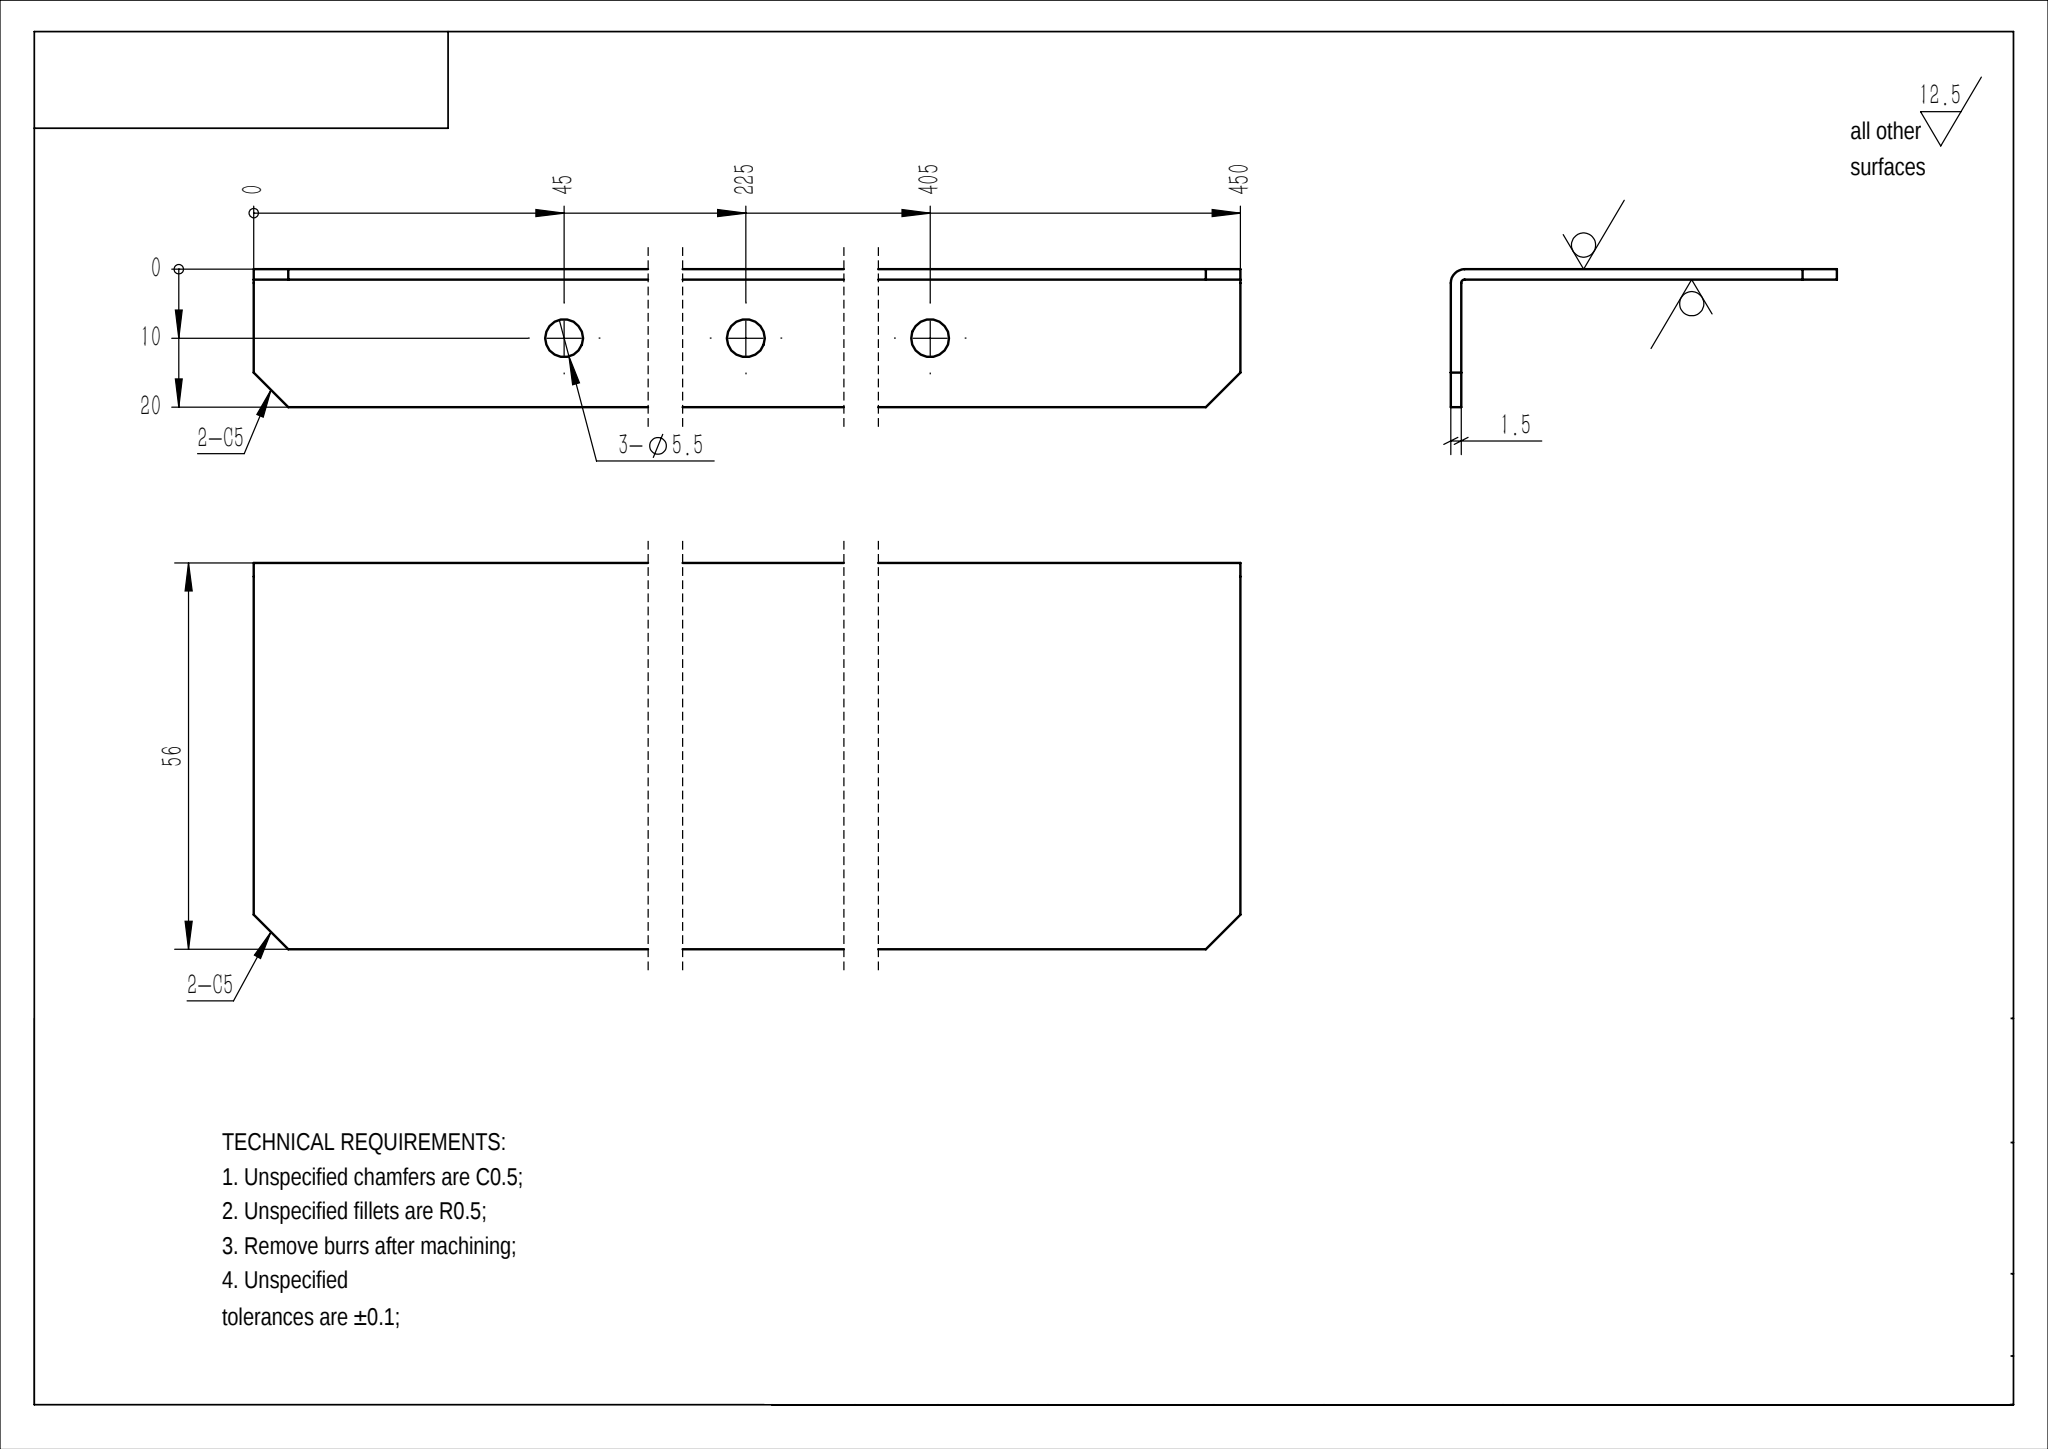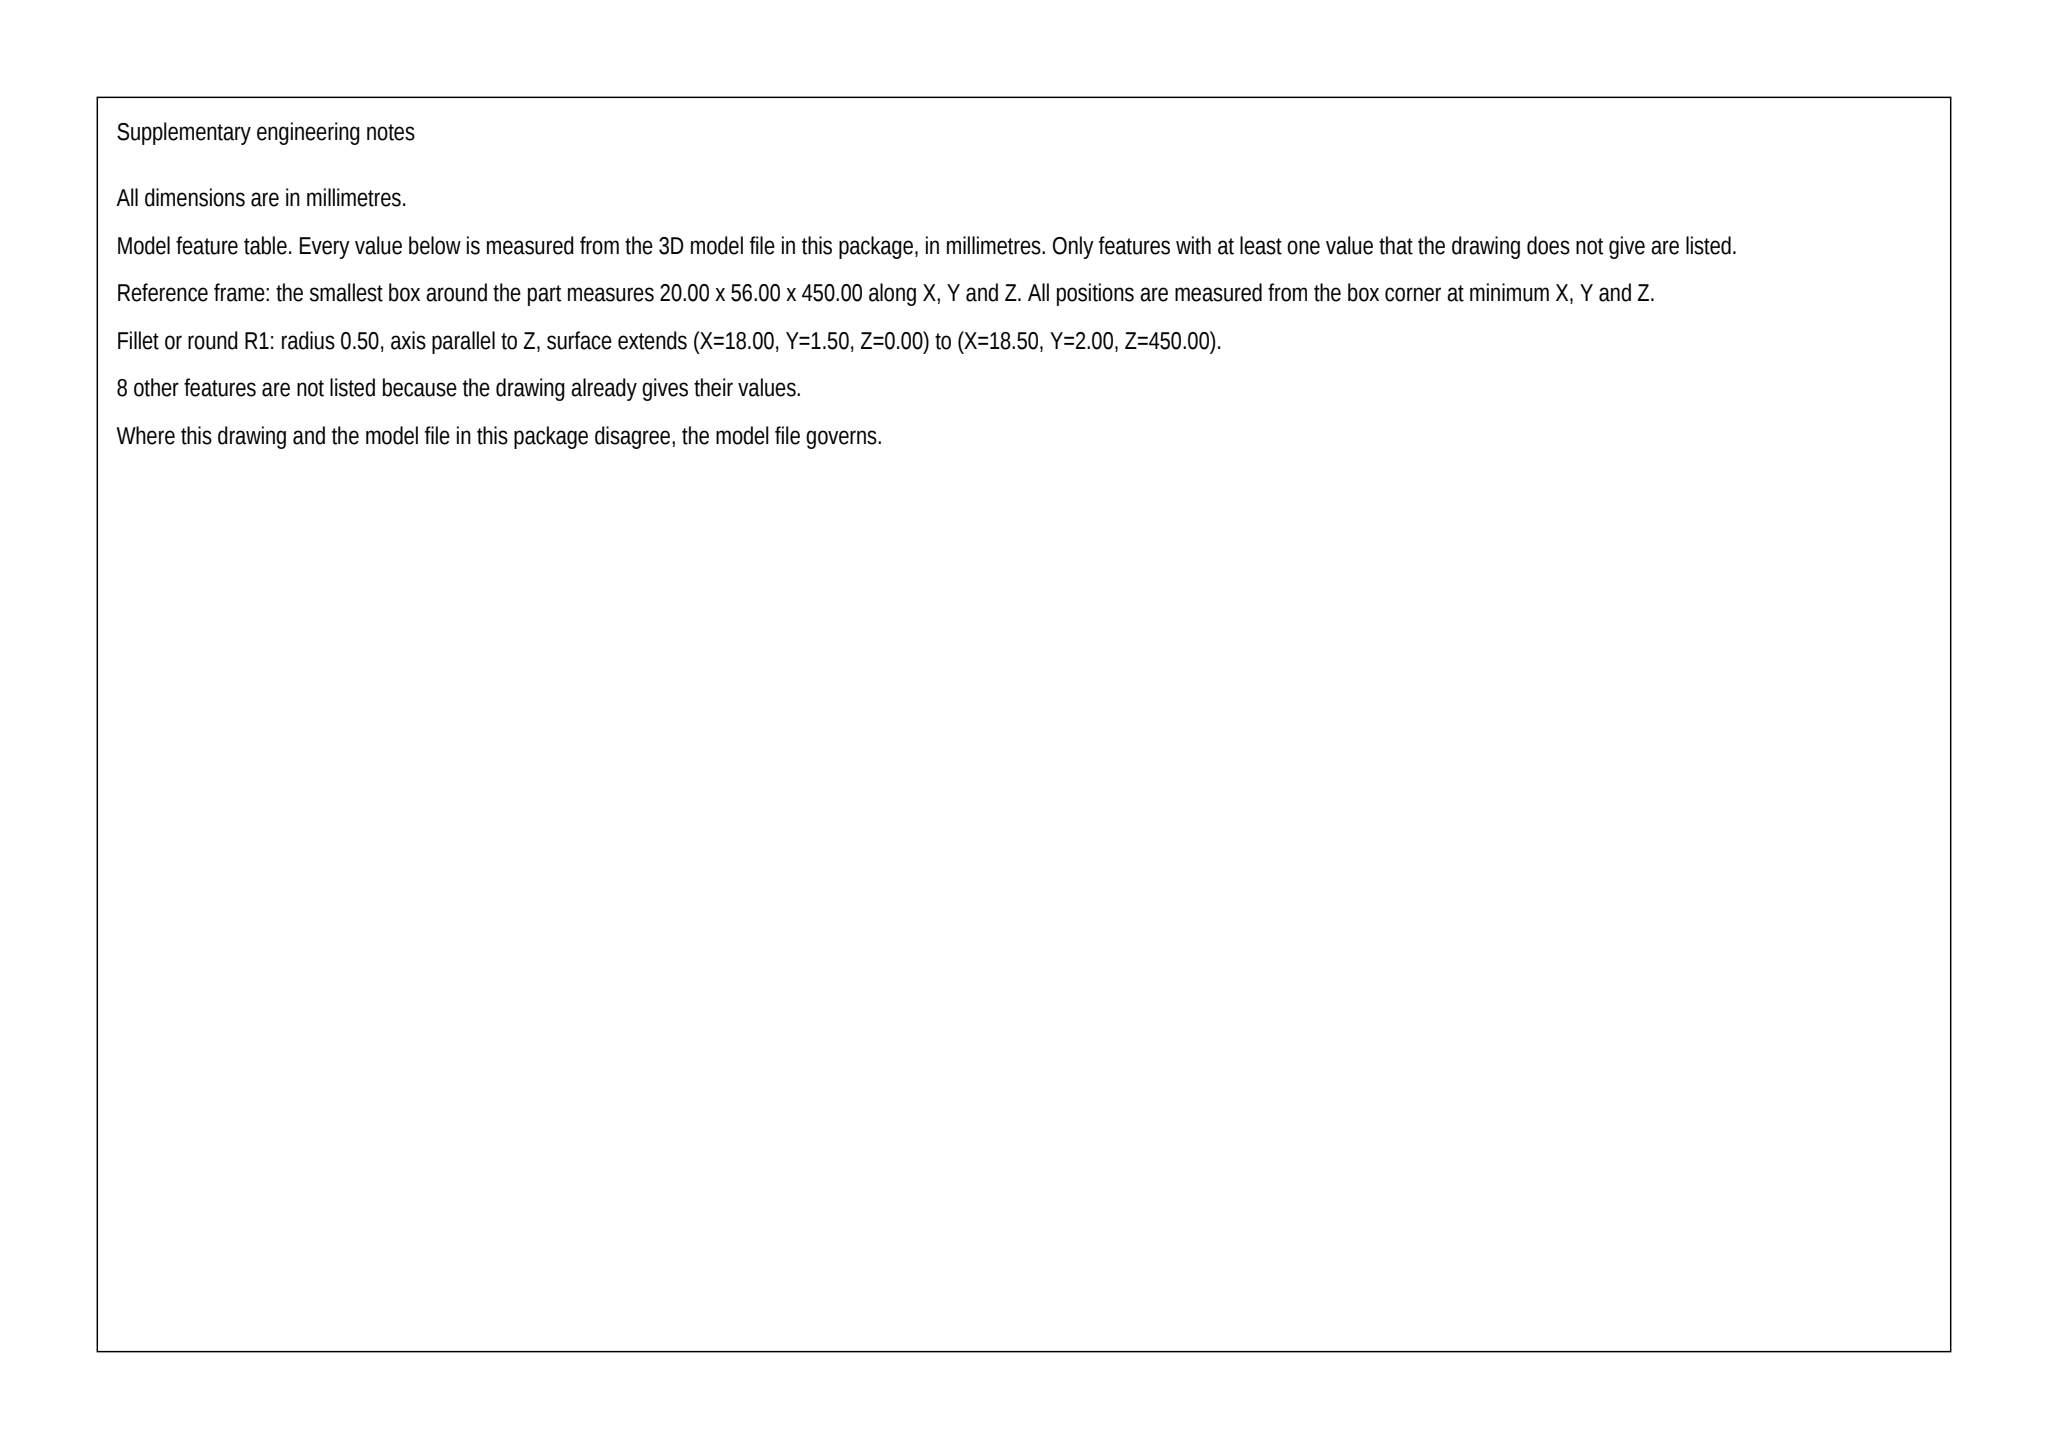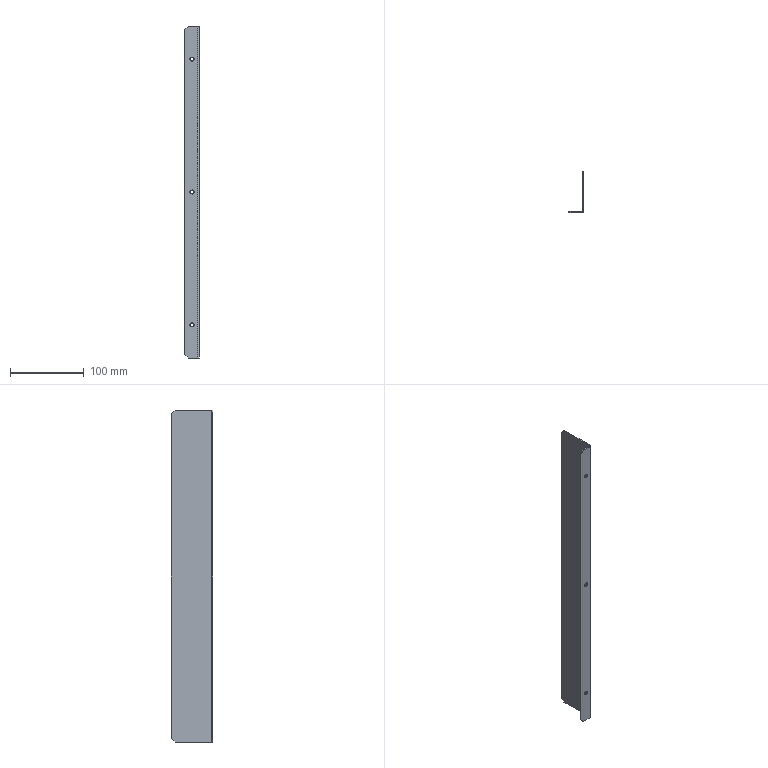Part | SolidWorks | mm | 1 solid | 24 faces | box 20 x 56 x 450 mm | volume 49743 mm3 | plane 16 | cylinder 8 | commonest cylinder face diameters 5.5 x6 1 x1 4 x1
STEP:
#1=CARTESIAN_POINT('',(-8.5,-1.5,-2.75));
#2=VERTEX_POINT('',#1);
#3=CARTESIAN_POINT('',(-8.5,-1.5,2.75));
#4=VERTEX_POINT('',#3);
#5=CARTESIAN_POINT('',(-8.5,-1.5,0.));
#6=DIRECTION('',(0.,1.,0.));
#7=DIRECTION('',(0.,0.,1.));
#8=AXIS2_PLACEMENT_3D('',#5,#6,#7);
#9=CIRCLE('',#8,2.75);
#10=EDGE_CURVE('',#2,#4,#9,.T.);
#11=ORIENTED_EDGE('',*,*,#10,.F.);
#12=CARTESIAN_POINT('',(-8.5,0.,-2.75));
#13=VERTEX_POINT('',#12);
#14=CARTESIAN_POINT('',(-8.5,-1.5,-2.75));
#15=DIRECTION('',(0.,1.,0.));
#16=VECTOR('',#15,1000.);
#17=LINE('',#14,#16);
#18=EDGE_CURVE('',#2,#13,#17,.T.);
#19=ORIENTED_EDGE('',*,*,#18,.T.);
#20=CARTESIAN_POINT('',(-8.5,0.,2.75));
#21=VERTEX_POINT('',#20);
#22=CARTESIAN_POINT('',(-8.5,0.,0.));
#23=DIRECTION('',(0.,1.,0.));
#24=DIRECTION('',(0.,0.,1.));
#25=AXIS2_PLACEMENT_3D('',#22,#23,#24);
#26=CIRCLE('',#25,2.75);
#27=EDGE_CURVE('',#13,#21,#26,.T.);
#28=ORIENTED_EDGE('',*,*,#27,.T.);
#29=CARTESIAN_POINT('',(-8.5,-1.5,2.75));
#30=DIRECTION('',(0.,1.,0.));
#31=VECTOR('',#30,1000.);
#32=LINE('',#29,#31);
#33=EDGE_CURVE('',#4,#21,#32,.T.);
#34=ORIENTED_EDGE('',*,*,#33,.F.);
#35=EDGE_LOOP('',(#11,#19,#28,#34));
#36=FACE_OUTER_BOUND('',#35,.T.);
#37=CARTESIAN_POINT('',(-8.5,-1.5,0.));
#38=DIRECTION('',(0.,1.,0.));
#39=DIRECTION('',(0.,0.,1.));
#40=AXIS2_PLACEMENT_3D('',#37,#38,#39);
#41=CYLINDRICAL_SURFACE('',#40,2.75);
#42=ADVANCED_FACE('',(#36),#41,.F.);
#43=CARTESIAN_POINT('',(-8.5,-1.5,177.25));
#44=VERTEX_POINT('',#43);
#45=CARTESIAN_POINT('',(-8.5,-1.5,182.75));
#46=VERTEX_POINT('',#45);
#47=CARTESIAN_POINT('',(-8.5,-1.5,180.));
#48=DIRECTION('',(0.,1.,0.));
#49=DIRECTION('',(0.,0.,-1.));
#50=AXIS2_PLACEMENT_3D('',#47,#48,#49);
#51=CIRCLE('',#50,2.75);
#52=EDGE_CURVE('',#44,#46,#51,.T.);
#53=ORIENTED_EDGE('',*,*,#52,.F.);
#54=CARTESIAN_POINT('',(-8.5,0.,177.25));
#55=VERTEX_POINT('',#54);
#56=CARTESIAN_POINT('',(-8.5,-1.5,177.25));
#57=DIRECTION('',(0.,1.,0.));
#58=VECTOR('',#57,1000.);
#59=LINE('',#56,#58);
#60=EDGE_CURVE('',#44,#55,#59,.T.);
#61=ORIENTED_EDGE('',*,*,#60,.T.);
#62=CARTESIAN_POINT('',(-8.5,0.,182.75));
#63=VERTEX_POINT('',#62);
#64=CARTESIAN_POINT('',(-8.5,0.,180.));
#65=DIRECTION('',(0.,1.,0.));
#66=DIRECTION('',(0.,0.,-1.));
#67=AXIS2_PLACEMENT_3D('',#64,#65,#66);
#68=CIRCLE('',#67,2.75);
#69=EDGE_CURVE('',#55,#63,#68,.T.);
#70=ORIENTED_EDGE('',*,*,#69,.T.);
#71=CARTESIAN_POINT('',(-8.5,-1.5,182.75));
#72=DIRECTION('',(0.,1.,0.));
#73=VECTOR('',#72,1000.);
#74=LINE('',#71,#73);
#75=EDGE_CURVE('',#46,#63,#74,.T.);
#76=ORIENTED_EDGE('',*,*,#75,.F.);
#77=EDGE_LOOP('',(#53,#61,#70,#76));
#78=FACE_OUTER_BOUND('',#77,.T.);
#79=CARTESIAN_POINT('',(-8.5,-1.5,180.));
#80=DIRECTION('',(0.,1.,0.));
#81=DIRECTION('',(0.,0.,1.));
#82=AXIS2_PLACEMENT_3D('',#79,#80,#81);
#83=CYLINDRICAL_SURFACE('',#82,2.75);
#84=ADVANCED_FACE('',(#78),#83,.F.);
#85=CARTESIAN_POINT('',(-8.5,-1.5,-182.75));
#86=VERTEX_POINT('',#85);
#87=CARTESIAN_POINT('',(-8.5,-1.5,-177.25));
#88=VERTEX_POINT('',#87);
#89=CARTESIAN_POINT('',(-8.5,-1.5,-180.));
#90=DIRECTION('',(0.,1.,0.));
#91=DIRECTION('',(0.,0.,1.));
#92=AXIS2_PLACEMENT_3D('',#89,#90,#91);
#93=CIRCLE('',#92,2.75);
#94=EDGE_CURVE('',#86,#88,#93,.T.);
#95=ORIENTED_EDGE('',*,*,#94,.F.);
#96=CARTESIAN_POINT('',(-8.5,0.,-182.75));
#97=VERTEX_POINT('',#96);
#98=CARTESIAN_POINT('',(-8.5,-1.5,-182.75));
#99=DIRECTION('',(0.,1.,0.));
#100=VECTOR('',#99,1000.);
#101=LINE('',#98,#100);
#102=EDGE_CURVE('',#86,#97,#101,.T.);
#103=ORIENTED_EDGE('',*,*,#102,.T.);
#104=CARTESIAN_POINT('',(-8.5,0.,-177.25));
#105=VERTEX_POINT('',#104);
#106=CARTESIAN_POINT('',(-8.5,0.,-180.));
#107=DIRECTION('',(0.,1.,0.));
#108=DIRECTION('',(0.,0.,1.));
#109=AXIS2_PLACEMENT_3D('',#106,#107,#108);
#110=CIRCLE('',#109,2.75);
#111=EDGE_CURVE('',#97,#105,#110,.T.);
#112=ORIENTED_EDGE('',*,*,#111,.T.);
#113=CARTESIAN_POINT('',(-8.5,-1.5,-177.25));
#114=DIRECTION('',(0.,1.,0.));
#115=VECTOR('',#114,1000.);
#116=LINE('',#113,#115);
#117=EDGE_CURVE('',#88,#105,#116,.T.);
#118=ORIENTED_EDGE('',*,*,#117,.F.);
#119=EDGE_LOOP('',(#95,#103,#112,#118));
#120=FACE_OUTER_BOUND('',#119,.T.);
#121=CARTESIAN_POINT('',(-8.5,-1.5,-180.));
#122=DIRECTION('',(0.,1.,0.));
#123=DIRECTION('',(0.,0.,1.));
#124=AXIS2_PLACEMENT_3D('',#121,#122,#123);
#125=CYLINDRICAL_SURFACE('',#124,2.75);
#126=ADVANCED_FACE('',(#120),#125,.F.);
#127=CARTESIAN_POINT('',(0.,0.5,225.));
#128=VERTEX_POINT('',#127);
#129=CARTESIAN_POINT('',(1.5,0.5,225.));
#130=VERTEX_POINT('',#129);
#131=CARTESIAN_POINT('',(0.,0.5,225.));
#132=DIRECTION('',(1.,0.,0.));
#133=VECTOR('',#132,1000.);
#134=LINE('',#131,#133);
#135=EDGE_CURVE('',#128,#130,#134,.T.);
#136=ORIENTED_EDGE('',*,*,#135,.F.);
#137=CARTESIAN_POINT('',(-0.5,0.,225.));
#138=VERTEX_POINT('',#137);
#139=CARTESIAN_POINT('',(-0.5,0.5,225.));
#140=DIRECTION('',(0.,0.,1.));
#141=DIRECTION('',(-1.,0.,0.));
#142=AXIS2_PLACEMENT_3D('',#139,#140,#141);
#143=CIRCLE('',#142,0.5);
#144=EDGE_CURVE('',#138,#128,#143,.T.);
#145=ORIENTED_EDGE('',*,*,#144,.F.);
#146=CARTESIAN_POINT('',(-0.5,-1.5,225.));
#147=VERTEX_POINT('',#146);
#148=CARTESIAN_POINT('',(-0.5,-1.5,225.));
#149=DIRECTION('',(0.,1.,0.));
#150=VECTOR('',#149,1000.);
#151=LINE('',#148,#150);
#152=EDGE_CURVE('',#147,#138,#151,.T.);
#153=ORIENTED_EDGE('',*,*,#152,.F.);
#154=CARTESIAN_POINT('',(-0.5,0.5,225.));
#155=DIRECTION('',(0.,0.,1.));
#156=DIRECTION('',(1.,0.,0.));
#157=AXIS2_PLACEMENT_3D('',#154,#155,#156);
#158=CIRCLE('',#157,2.);
#159=EDGE_CURVE('',#147,#130,#158,.T.);
#160=ORIENTED_EDGE('',*,*,#159,.T.);
#161=EDGE_LOOP('',(#136,#145,#153,#160));
#162=FACE_OUTER_BOUND('',#161,.T.);
#163=CARTESIAN_POINT('',(0.,0.5,225.));
#164=DIRECTION('',(0.,0.,1.));
#165=DIRECTION('',(1.,0.,0.));
#166=AXIS2_PLACEMENT_3D('',#163,#164,#165);
#167=PLANE('',#166);
#168=ADVANCED_FACE('',(#162),#167,.T.);
#169=CARTESIAN_POINT('',(1.5,49.5,225.));
#170=VERTEX_POINT('',#169);
#171=CARTESIAN_POINT('',(1.5,0.,225.));
#172=DIRECTION('',(0.,1.,0.));
#173=VECTOR('',#172,1000.);
#174=LINE('',#171,#173);
#175=EDGE_CURVE('',#130,#170,#174,.T.);
#176=ORIENTED_EDGE('',*,*,#175,.T.);
#177=CARTESIAN_POINT('',(0.,49.5,225.));
#178=VERTEX_POINT('',#177);
#179=CARTESIAN_POINT('',(-0.5,49.5,225.));
#180=DIRECTION('',(-1.,0.,0.));
#181=VECTOR('',#180,1000.);
#182=LINE('',#179,#181);
#183=EDGE_CURVE('',#170,#178,#182,.T.);
#184=ORIENTED_EDGE('',*,*,#183,.T.);
#185=CARTESIAN_POINT('',(0.,0.,225.));
#186=DIRECTION('',(0.,1.,0.));
#187=VECTOR('',#186,1000.);
#188=LINE('',#185,#187);
#189=EDGE_CURVE('',#128,#178,#188,.T.);
#190=ORIENTED_EDGE('',*,*,#189,.F.);
#191=ORIENTED_EDGE('',*,*,#135,.T.);
#192=EDGE_LOOP('',(#176,#184,#190,#191));
#193=FACE_OUTER_BOUND('',#192,.T.);
#194=CARTESIAN_POINT('',(-0.5,-1.5,225.));
#195=DIRECTION('',(0.,0.,1.));
#196=DIRECTION('',(1.,0.,0.));
#197=AXIS2_PLACEMENT_3D('',#194,#195,#196);
#198=PLANE('',#197);
#199=ADVANCED_FACE('',(#193),#198,.T.);
#200=CARTESIAN_POINT('',(-0.5,0.,-225.));
#201=VERTEX_POINT('',#200);
#202=CARTESIAN_POINT('',(-0.5,-1.5,-225.));
#203=VERTEX_POINT('',#202);
#204=CARTESIAN_POINT('',(-0.5,0.,-225.));
#205=DIRECTION('',(-0.,-1.,0.));
#206=VECTOR('',#205,1000.);
#207=LINE('',#204,#206);
#208=EDGE_CURVE('',#201,#203,#207,.T.);
#209=ORIENTED_EDGE('',*,*,#208,.F.);
#210=CARTESIAN_POINT('',(0.,0.5,-225.));
#211=VERTEX_POINT('',#210);
#212=CARTESIAN_POINT('',(-0.5,0.5,-225.));
#213=DIRECTION('',(0.,0.,1.));
#214=DIRECTION('',(-1.,0.,0.));
#215=AXIS2_PLACEMENT_3D('',#212,#213,#214);
#216=CIRCLE('',#215,0.5);
#217=EDGE_CURVE('',#201,#211,#216,.T.);
#218=ORIENTED_EDGE('',*,*,#217,.T.);
#219=CARTESIAN_POINT('',(1.5,0.5,-225.));
#220=VERTEX_POINT('',#219);
#221=CARTESIAN_POINT('',(1.5,0.5,-225.));
#222=DIRECTION('',(-1.,0.,0.));
#223=VECTOR('',#222,1000.);
#224=LINE('',#221,#223);
#225=EDGE_CURVE('',#220,#211,#224,.T.);
#226=ORIENTED_EDGE('',*,*,#225,.F.);
#227=CARTESIAN_POINT('',(-0.5,0.5,-225.));
#228=DIRECTION('',(0.,0.,1.));
#229=DIRECTION('',(1.,0.,0.));
#230=AXIS2_PLACEMENT_3D('',#227,#228,#229);
#231=CIRCLE('',#230,2.);
#232=EDGE_CURVE('',#203,#220,#231,.T.);
#233=ORIENTED_EDGE('',*,*,#232,.F.);
#234=EDGE_LOOP('',(#209,#218,#226,#233));
#235=FACE_OUTER_BOUND('',#234,.T.);
#236=CARTESIAN_POINT('',(-0.5,0.,-225.));
#237=DIRECTION('',(0.,0.,-1.));
#238=DIRECTION('',(-1.,0.,0.));
#239=AXIS2_PLACEMENT_3D('',#236,#237,#238);
#240=PLANE('',#239);
#241=ADVANCED_FACE('',(#235),#240,.T.);
#242=CARTESIAN_POINT('',(-13.5,-1.5,-225.));
#243=VERTEX_POINT('',#242);
#244=CARTESIAN_POINT('',(-18.5,-1.5,-225.));
#245=DIRECTION('',(1.,0.,0.));
#246=VECTOR('',#245,1000.);
#247=LINE('',#244,#246);
#248=EDGE_CURVE('',#243,#203,#247,.T.);
#249=ORIENTED_EDGE('',*,*,#248,.F.);
#250=CARTESIAN_POINT('',(-13.5,0.,-225.));
#251=VERTEX_POINT('',#250);
#252=CARTESIAN_POINT('',(-13.5,0.5,-225.));
#253=DIRECTION('',(0.,1.,0.));
#254=VECTOR('',#253,1000.);
#255=LINE('',#252,#254);
#256=EDGE_CURVE('',#243,#251,#255,.T.);
#257=ORIENTED_EDGE('',*,*,#256,.T.);
#258=CARTESIAN_POINT('',(-18.5,0.,-225.));
#259=DIRECTION('',(1.,0.,0.));
#260=VECTOR('',#259,1000.);
#261=LINE('',#258,#260);
#262=EDGE_CURVE('',#251,#201,#261,.T.);
#263=ORIENTED_EDGE('',*,*,#262,.T.);
#264=ORIENTED_EDGE('',*,*,#208,.T.);
#265=EDGE_LOOP('',(#249,#257,#263,#264));
#266=FACE_OUTER_BOUND('',#265,.T.);
#267=CARTESIAN_POINT('',(1.5,0.5,-225.));
#268=DIRECTION('',(0.,0.,-1.));
#269=DIRECTION('',(-1.,0.,0.));
#270=AXIS2_PLACEMENT_3D('',#267,#268,#269);
#271=PLANE('',#270);
#272=ADVANCED_FACE('',(#266),#271,.T.);
#273=CARTESIAN_POINT('',(1.5,54.5,220.));
#274=VERTEX_POINT('',#273);
#275=CARTESIAN_POINT('',(1.5,54.5,-220.));
#276=VERTEX_POINT('',#275);
#277=CARTESIAN_POINT('',(1.5,54.5,225.));
#278=DIRECTION('',(0.,0.,-1.));
#279=VECTOR('',#278,1000.);
#280=LINE('',#277,#279);
#281=EDGE_CURVE('',#274,#276,#280,.T.);
#282=ORIENTED_EDGE('',*,*,#281,.F.);
#283=CARTESIAN_POINT('',(1.5,54.5,220.));
#284=DIRECTION('',(0.,-0.7071,0.7071));
#285=VECTOR('',#284,1000.);
#286=LINE('',#283,#285);
#287=EDGE_CURVE('',#274,#170,#286,.T.);
#288=ORIENTED_EDGE('',*,*,#287,.T.);
#289=ORIENTED_EDGE('',*,*,#175,.F.);
#290=CARTESIAN_POINT('',(1.5,0.5,225.));
#291=DIRECTION('',(0.,0.,-1.));
#292=VECTOR('',#291,1000.);
#293=LINE('',#290,#292);
#294=EDGE_CURVE('',#130,#220,#293,.T.);
#295=ORIENTED_EDGE('',*,*,#294,.T.);
#296=CARTESIAN_POINT('',(1.5,49.5,-225.));
#297=VERTEX_POINT('',#296);
#298=CARTESIAN_POINT('',(1.5,0.,-225.));
#299=DIRECTION('',(0.,1.,0.));
#300=VECTOR('',#299,1000.);
#301=LINE('',#298,#300);
#302=EDGE_CURVE('',#220,#297,#301,.T.);
#303=ORIENTED_EDGE('',*,*,#302,.T.);
#304=CARTESIAN_POINT('',(1.5,49.5,-225.));
#305=DIRECTION('',(0.,0.7071,0.7071));
#306=VECTOR('',#305,1000.);
#307=LINE('',#304,#306);
#308=EDGE_CURVE('',#297,#276,#307,.T.);
#309=ORIENTED_EDGE('',*,*,#308,.T.);
#310=EDGE_LOOP('',(#282,#288,#289,#295,#303,#309));
#311=FACE_OUTER_BOUND('',#310,.T.);
#312=CARTESIAN_POINT('',(1.5,0.,225.));
#313=DIRECTION('',(-1.,0.,0.));
#314=DIRECTION('',(0.,0.,1.));
#315=AXIS2_PLACEMENT_3D('',#312,#313,#314);
#316=PLANE('',#315);
#317=ADVANCED_FACE('',(#311),#316,.F.);
#318=CARTESIAN_POINT('',(0.,54.5,220.));
#319=VERTEX_POINT('',#318);
#320=CARTESIAN_POINT('',(0.,54.5,-220.));
#321=VERTEX_POINT('',#320);
#322=CARTESIAN_POINT('',(0.,54.5,225.));
#323=DIRECTION('',(0.,0.,-1.));
#324=VECTOR('',#323,1000.);
#325=LINE('',#322,#324);
#326=EDGE_CURVE('',#319,#321,#325,.T.);
#327=ORIENTED_EDGE('',*,*,#326,.F.);
#328=CARTESIAN_POINT('',(0.,54.5,220.));
#329=DIRECTION('',(1.,0.,0.));
#330=VECTOR('',#329,1000.);
#331=LINE('',#328,#330);
#332=EDGE_CURVE('',#319,#274,#331,.T.);
#333=ORIENTED_EDGE('',*,*,#332,.T.);
#334=ORIENTED_EDGE('',*,*,#281,.T.);
#335=CARTESIAN_POINT('',(0.,54.5,-220.));
#336=DIRECTION('',(-1.,0.,0.));
#337=VECTOR('',#336,1000.);
#338=LINE('',#335,#337);
#339=EDGE_CURVE('',#276,#321,#338,.T.);
#340=ORIENTED_EDGE('',*,*,#339,.T.);
#341=EDGE_LOOP('',(#327,#333,#334,#340));
#342=FACE_OUTER_BOUND('',#341,.T.);
#343=CARTESIAN_POINT('',(0.,54.5,225.));
#344=DIRECTION('',(0.,1.,0.));
#345=DIRECTION('',(0.,0.,1.));
#346=AXIS2_PLACEMENT_3D('',#343,#344,#345);
#347=PLANE('',#346);
#348=ADVANCED_FACE('',(#342),#347,.T.);
#349=ORIENTED_EDGE('',*,*,#189,.T.);
#350=CARTESIAN_POINT('',(0.,24.75,249.75));
#351=DIRECTION('',(0.,0.7071,-0.7071));
#352=VECTOR('',#351,1000.);
#353=LINE('',#350,#352);
#354=EDGE_CURVE('',#178,#319,#353,.T.);
#355=ORIENTED_EDGE('',*,*,#354,.T.);
#356=ORIENTED_EDGE('',*,*,#326,.T.);
#357=CARTESIAN_POINT('',(0.,49.5,-225.));
#358=VERTEX_POINT('',#357);
#359=CARTESIAN_POINT('',(0.,249.75,-24.75));
#360=DIRECTION('',(0.,-0.7071,-0.7071));
#361=VECTOR('',#360,1000.);
#362=LINE('',#359,#361);
#363=EDGE_CURVE('',#321,#358,#362,.T.);
#364=ORIENTED_EDGE('',*,*,#363,.T.);
#365=CARTESIAN_POINT('',(0.,0.,-225.));
#366=DIRECTION('',(0.,1.,0.));
#367=VECTOR('',#366,1000.);
#368=LINE('',#365,#367);
#369=EDGE_CURVE('',#211,#358,#368,.T.);
#370=ORIENTED_EDGE('',*,*,#369,.F.);
#371=CARTESIAN_POINT('',(0.,0.5,225.));
#372=DIRECTION('',(0.,0.,-1.));
#373=VECTOR('',#372,1000.);
#374=LINE('',#371,#373);
#375=EDGE_CURVE('',#128,#211,#374,.T.);
#376=ORIENTED_EDGE('',*,*,#375,.F.);
#377=EDGE_LOOP('',(#349,#355,#356,#364,#370,#376));
#378=FACE_OUTER_BOUND('',#377,.T.);
#379=CARTESIAN_POINT('',(0.,0.,225.));
#380=DIRECTION('',(-1.,0.,0.));
#381=DIRECTION('',(0.,0.,1.));
#382=AXIS2_PLACEMENT_3D('',#379,#380,#381);
#383=PLANE('',#382);
#384=ADVANCED_FACE('',(#378),#383,.T.);
#385=ORIENTED_EDGE('',*,*,#217,.F.);
#386=CARTESIAN_POINT('',(-0.5,0.,225.));
#387=DIRECTION('',(0.,0.,-1.));
#388=VECTOR('',#387,1000.);
#389=LINE('',#386,#388);
#390=EDGE_CURVE('',#138,#201,#389,.T.);
#391=ORIENTED_EDGE('',*,*,#390,.F.);
#392=ORIENTED_EDGE('',*,*,#144,.T.);
#393=ORIENTED_EDGE('',*,*,#375,.T.);
#394=EDGE_LOOP('',(#385,#391,#392,#393));
#395=FACE_OUTER_BOUND('',#394,.T.);
#396=CARTESIAN_POINT('',(-0.5,0.5,225.));
#397=DIRECTION('',(0.,0.,-1.));
#398=DIRECTION('',(-1.,0.,0.));
#399=AXIS2_PLACEMENT_3D('',#396,#397,#398);
#400=CYLINDRICAL_SURFACE('',#399,0.5);
#401=ADVANCED_FACE('',(#395),#400,.F.);
#402=CARTESIAN_POINT('',(-8.5,0.,0.));
#403=DIRECTION('',(0.,1.,0.));
#404=DIRECTION('',(0.,0.,1.));
#405=AXIS2_PLACEMENT_3D('',#402,#403,#404);
#406=CIRCLE('',#405,2.75);
#407=EDGE_CURVE('',#21,#13,#406,.T.);
#408=ORIENTED_EDGE('',*,*,#407,.F.);
#409=ORIENTED_EDGE('',*,*,#27,.F.);
#410=EDGE_LOOP('',(#408,#409));
#411=FACE_BOUND('',#410,.T.);
#412=CARTESIAN_POINT('',(-8.5,0.,180.));
#413=DIRECTION('',(0.,1.,0.));
#414=DIRECTION('',(0.,0.,-1.));
#415=AXIS2_PLACEMENT_3D('',#412,#413,#414);
#416=CIRCLE('',#415,2.75);
#417=EDGE_CURVE('',#63,#55,#416,.T.);
#418=ORIENTED_EDGE('',*,*,#417,.F.);
#419=ORIENTED_EDGE('',*,*,#69,.F.);
#420=EDGE_LOOP('',(#418,#419));
#421=FACE_BOUND('',#420,.T.);
#422=CARTESIAN_POINT('',(-8.5,0.,-180.));
#423=DIRECTION('',(0.,1.,0.));
#424=DIRECTION('',(0.,0.,1.));
#425=AXIS2_PLACEMENT_3D('',#422,#423,#424);
#426=CIRCLE('',#425,2.75);
#427=EDGE_CURVE('',#105,#97,#426,.T.);
#428=ORIENTED_EDGE('',*,*,#427,.F.);
#429=ORIENTED_EDGE('',*,*,#111,.F.);
#430=EDGE_LOOP('',(#428,#429));
#431=FACE_BOUND('',#430,.T.);
#432=CARTESIAN_POINT('',(-18.5,0.,220.));
#433=VERTEX_POINT('',#432);
#434=CARTESIAN_POINT('',(-18.5,0.,-220.));
#435=VERTEX_POINT('',#434);
#436=CARTESIAN_POINT('',(-18.5,0.,225.));
#437=DIRECTION('',(0.,0.,-1.));
#438=VECTOR('',#437,1000.);
#439=LINE('',#436,#438);
#440=EDGE_CURVE('',#433,#435,#439,.T.);
#441=ORIENTED_EDGE('',*,*,#440,.F.);
#442=CARTESIAN_POINT('',(-13.5,0.,225.));
#443=VERTEX_POINT('',#442);
#444=CARTESIAN_POINT('',(-16.,0.,222.5));
#445=DIRECTION('',(0.7071,0.,0.7071));
#446=VECTOR('',#445,1000.);
#447=LINE('',#444,#446);
#448=EDGE_CURVE('',#433,#443,#447,.T.);
#449=ORIENTED_EDGE('',*,*,#448,.T.);
#450=CARTESIAN_POINT('',(-18.5,0.,225.));
#451=DIRECTION('',(1.,0.,0.));
#452=VECTOR('',#451,1000.);
#453=LINE('',#450,#452);
#454=EDGE_CURVE('',#443,#138,#453,.T.);
#455=ORIENTED_EDGE('',*,*,#454,.T.);
#456=ORIENTED_EDGE('',*,*,#390,.T.);
#457=ORIENTED_EDGE('',*,*,#262,.F.);
#458=CARTESIAN_POINT('',(-241.,0.,2.5));
#459=DIRECTION('',(-0.7071,0.,0.7071));
#460=VECTOR('',#459,1000.);
#461=LINE('',#458,#460);
#462=EDGE_CURVE('',#251,#435,#461,.T.);
#463=ORIENTED_EDGE('',*,*,#462,.T.);
#464=EDGE_LOOP('',(#441,#449,#455,#456,#457,#463));
#465=FACE_OUTER_BOUND('',#464,.T.);
#466=CARTESIAN_POINT('',(-18.5,0.,225.));
#467=DIRECTION('',(0.,1.,0.));
#468=DIRECTION('',(0.,0.,1.));
#469=AXIS2_PLACEMENT_3D('',#466,#467,#468);
#470=PLANE('',#469);
#471=ADVANCED_FACE('',(#411,#421,#431,#465),#470,.T.);
#472=CARTESIAN_POINT('',(-18.5,-1.5,220.));
#473=VERTEX_POINT('',#472);
#474=CARTESIAN_POINT('',(-18.5,-1.5,-220.));
#475=VERTEX_POINT('',#474);
#476=CARTESIAN_POINT('',(-18.5,-1.5,225.));
#477=DIRECTION('',(0.,0.,-1.));
#478=VECTOR('',#477,1000.);
#479=LINE('',#476,#478);
#480=EDGE_CURVE('',#473,#475,#479,.T.);
#481=ORIENTED_EDGE('',*,*,#480,.F.);
#482=CARTESIAN_POINT('',(-18.5,0.,220.));
#483=DIRECTION('',(0.,1.,0.));
#484=VECTOR('',#483,1000.);
#485=LINE('',#482,#484);
#486=EDGE_CURVE('',#473,#433,#485,.T.);
#487=ORIENTED_EDGE('',*,*,#486,.T.);
#488=ORIENTED_EDGE('',*,*,#440,.T.);
#489=CARTESIAN_POINT('',(-18.5,-1.5,-220.));
#490=DIRECTION('',(0.,-1.,0.));
#491=VECTOR('',#490,1000.);
#492=LINE('',#489,#491);
#493=EDGE_CURVE('',#435,#475,#492,.T.);
#494=ORIENTED_EDGE('',*,*,#493,.T.);
#495=EDGE_LOOP('',(#481,#487,#488,#494));
#496=FACE_OUTER_BOUND('',#495,.T.);
#497=CARTESIAN_POINT('',(-18.5,-1.5,225.));
#498=DIRECTION('',(-1.,0.,0.));
#499=DIRECTION('',(0.,0.,1.));
#500=AXIS2_PLACEMENT_3D('',#497,#498,#499);
#501=PLANE('',#500);
#502=ADVANCED_FACE('',(#496),#501,.T.);
#503=CARTESIAN_POINT('',(-8.5,-1.5,0.));
#504=DIRECTION('',(0.,1.,0.));
#505=DIRECTION('',(0.,0.,1.));
#506=AXIS2_PLACEMENT_3D('',#503,#504,#505);
#507=CIRCLE('',#506,2.75);
#508=EDGE_CURVE('',#4,#2,#507,.T.);
#509=ORIENTED_EDGE('',*,*,#508,.T.);
#510=ORIENTED_EDGE('',*,*,#10,.T.);
#511=EDGE_LOOP('',(#509,#510));
#512=FACE_BOUND('',#511,.T.);
#513=CARTESIAN_POINT('',(-8.5,-1.5,180.));
#514=DIRECTION('',(0.,1.,0.));
#515=DIRECTION('',(0.,0.,-1.));
#516=AXIS2_PLACEMENT_3D('',#513,#514,#515);
#517=CIRCLE('',#516,2.75);
#518=EDGE_CURVE('',#46,#44,#517,.T.);
#519=ORIENTED_EDGE('',*,*,#518,.T.);
#520=ORIENTED_EDGE('',*,*,#52,.T.);
#521=EDGE_LOOP('',(#519,#520));
#522=FACE_BOUND('',#521,.T.);
#523=CARTESIAN_POINT('',(-8.5,-1.5,-180.));
#524=DIRECTION('',(0.,1.,0.));
#525=DIRECTION('',(0.,0.,1.));
#526=AXIS2_PLACEMENT_3D('',#523,#524,#525);
#527=CIRCLE('',#526,2.75);
#528=EDGE_CURVE('',#88,#86,#527,.T.);
#529=ORIENTED_EDGE('',*,*,#528,.T.);
#530=ORIENTED_EDGE('',*,*,#94,.T.);
#531=EDGE_LOOP('',(#529,#530));
#532=FACE_BOUND('',#531,.T.);
#533=CARTESIAN_POINT('',(-13.5,-1.5,225.));
#534=VERTEX_POINT('',#533);
#535=CARTESIAN_POINT('',(-18.5,-1.5,225.));
#536=DIRECTION('',(1.,0.,0.));
#537=VECTOR('',#536,1000.);
#538=LINE('',#535,#537);
#539=EDGE_CURVE('',#534,#147,#538,.T.);
#540=ORIENTED_EDGE('',*,*,#539,.F.);
#541=CARTESIAN_POINT('',(-18.5,-1.5,220.));
#542=DIRECTION('',(-0.7071,0.,-0.7071));
#543=VECTOR('',#542,1000.);
#544=LINE('',#541,#543);
#545=EDGE_CURVE('',#534,#473,#544,.T.);
#546=ORIENTED_EDGE('',*,*,#545,.T.);
#547=ORIENTED_EDGE('',*,*,#480,.T.);
#548=CARTESIAN_POINT('',(-13.5,-1.5,-225.));
#549=DIRECTION('',(0.7071,0.,-0.7071));
#550=VECTOR('',#549,1000.);
#551=LINE('',#548,#550);
#552=EDGE_CURVE('',#475,#243,#551,.T.);
#553=ORIENTED_EDGE('',*,*,#552,.T.);
#554=ORIENTED_EDGE('',*,*,#248,.T.);
#555=CARTESIAN_POINT('',(-0.5,-1.5,225.));
#556=DIRECTION('',(0.,0.,-1.));
#557=VECTOR('',#556,1000.);
#558=LINE('',#555,#557);
#559=EDGE_CURVE('',#147,#203,#558,.T.);
#560=ORIENTED_EDGE('',*,*,#559,.F.);
#561=EDGE_LOOP('',(#540,#546,#547,#553,#554,#560));
#562=FACE_OUTER_BOUND('',#561,.T.);
#563=CARTESIAN_POINT('',(-18.5,-1.5,225.));
#564=DIRECTION('',(0.,1.,0.));
#565=DIRECTION('',(0.,0.,1.));
#566=AXIS2_PLACEMENT_3D('',#563,#564,#565);
#567=PLANE('',#566);
#568=ADVANCED_FACE('',(#512,#522,#532,#562),#567,.F.);
#569=ORIENTED_EDGE('',*,*,#232,.T.);
#570=ORIENTED_EDGE('',*,*,#294,.F.);
#571=ORIENTED_EDGE('',*,*,#159,.F.);
#572=ORIENTED_EDGE('',*,*,#559,.T.);
#573=EDGE_LOOP('',(#569,#570,#571,#572));
#574=FACE_OUTER_BOUND('',#573,.T.);
#575=CARTESIAN_POINT('',(-0.5,0.5,225.));
#576=DIRECTION('',(0.,0.,-1.));
#577=DIRECTION('',(-1.,0.,0.));
#578=AXIS2_PLACEMENT_3D('',#575,#576,#577);
#579=CYLINDRICAL_SURFACE('',#578,2.);
#580=ADVANCED_FACE('',(#574),#579,.T.);
#581=ORIENTED_EDGE('',*,*,#454,.F.);
#582=CARTESIAN_POINT('',(-13.5,-1.5,225.));
#583=DIRECTION('',(0.,-1.,0.));
#584=VECTOR('',#583,1000.);
#585=LINE('',#582,#584);
#586=EDGE_CURVE('',#443,#534,#585,.T.);
#587=ORIENTED_EDGE('',*,*,#586,.T.);
#588=ORIENTED_EDGE('',*,*,#539,.T.);
#589=ORIENTED_EDGE('',*,*,#152,.T.);
#590=EDGE_LOOP('',(#581,#587,#588,#589));
#591=FACE_OUTER_BOUND('',#590,.T.);
#592=CARTESIAN_POINT('',(-0.5,0.5,225.));
#593=DIRECTION('',(0.,0.,-1.));
#594=DIRECTION('',(-1.,0.,0.));
#595=AXIS2_PLACEMENT_3D('',#592,#593,#594);
#596=PLANE('',#595);
#597=ADVANCED_FACE('',(#591),#596,.F.);
#598=ORIENTED_EDGE('',*,*,#369,.T.);
#599=CARTESIAN_POINT('',(-0.5,49.5,-225.));
#600=DIRECTION('',(1.,0.,0.));
#601=VECTOR('',#600,1000.);
#602=LINE('',#599,#601);
#603=EDGE_CURVE('',#358,#297,#602,.T.);
#604=ORIENTED_EDGE('',*,*,#603,.T.);
#605=ORIENTED_EDGE('',*,*,#302,.F.);
#606=ORIENTED_EDGE('',*,*,#225,.T.);
#607=EDGE_LOOP('',(#598,#604,#605,#606));
#608=FACE_OUTER_BOUND('',#607,.T.);
#609=CARTESIAN_POINT('',(-0.5,0.5,-225.));
#610=DIRECTION('',(0.,0.,-1.));
#611=DIRECTION('',(-1.,0.,0.));
#612=AXIS2_PLACEMENT_3D('',#609,#610,#611);
#613=PLANE('',#612);
#614=ADVANCED_FACE('',(#608),#613,.T.);
#615=ORIENTED_EDGE('',*,*,#102,.F.);
#616=ORIENTED_EDGE('',*,*,#528,.F.);
#617=ORIENTED_EDGE('',*,*,#117,.T.);
#618=ORIENTED_EDGE('',*,*,#427,.T.);
#619=EDGE_LOOP('',(#615,#616,#617,#618));
#620=FACE_OUTER_BOUND('',#619,.T.);
#621=CARTESIAN_POINT('',(-8.5,-1.5,-180.));
#622=DIRECTION('',(0.,1.,0.));
#623=DIRECTION('',(0.,0.,1.));
#624=AXIS2_PLACEMENT_3D('',#621,#622,#623);
#625=CYLINDRICAL_SURFACE('',#624,2.75);
#626=ADVANCED_FACE('',(#620),#625,.F.);
#627=ORIENTED_EDGE('',*,*,#60,.F.);
#628=ORIENTED_EDGE('',*,*,#518,.F.);
#629=ORIENTED_EDGE('',*,*,#75,.T.);
#630=ORIENTED_EDGE('',*,*,#417,.T.);
#631=EDGE_LOOP('',(#627,#628,#629,#630));
#632=FACE_OUTER_BOUND('',#631,.T.);
#633=CARTESIAN_POINT('',(-8.5,-1.5,180.));
#634=DIRECTION('',(0.,1.,0.));
#635=DIRECTION('',(0.,0.,1.));
#636=AXIS2_PLACEMENT_3D('',#633,#634,#635);
#637=CYLINDRICAL_SURFACE('',#636,2.75);
#638=ADVANCED_FACE('',(#632),#637,.F.);
#639=ORIENTED_EDGE('',*,*,#18,.F.);
#640=ORIENTED_EDGE('',*,*,#508,.F.);
#641=ORIENTED_EDGE('',*,*,#33,.T.);
#642=ORIENTED_EDGE('',*,*,#407,.T.);
#643=EDGE_LOOP('',(#639,#640,#641,#642));
#644=FACE_OUTER_BOUND('',#643,.T.);
#645=CARTESIAN_POINT('',(-8.5,-1.5,0.));
#646=DIRECTION('',(0.,1.,0.));
#647=DIRECTION('',(0.,0.,1.));
#648=AXIS2_PLACEMENT_3D('',#645,#646,#647);
#649=CYLINDRICAL_SURFACE('',#648,2.75);
#650=ADVANCED_FACE('',(#644),#649,.F.);
#651=ORIENTED_EDGE('',*,*,#354,.F.);
#652=ORIENTED_EDGE('',*,*,#183,.F.);
#653=ORIENTED_EDGE('',*,*,#287,.F.);
#654=ORIENTED_EDGE('',*,*,#332,.F.);
#655=EDGE_LOOP('',(#651,#652,#653,#654));
#656=FACE_OUTER_BOUND('',#655,.T.);
#657=CARTESIAN_POINT('',(0.,54.5,220.));
#658=DIRECTION('',(0.,-0.7071,-0.7071));
#659=DIRECTION('',(1.,0.,0.));
#660=AXIS2_PLACEMENT_3D('',#657,#658,#659);
#661=PLANE('',#660);
#662=ADVANCED_FACE('',(#656),#661,.F.);
#663=ORIENTED_EDGE('',*,*,#545,.F.);
#664=ORIENTED_EDGE('',*,*,#586,.F.);
#665=ORIENTED_EDGE('',*,*,#448,.F.);
#666=ORIENTED_EDGE('',*,*,#486,.F.);
#667=EDGE_LOOP('',(#663,#664,#665,#666));
#668=FACE_OUTER_BOUND('',#667,.T.);
#669=CARTESIAN_POINT('',(-18.5,-1.5,220.));
#670=DIRECTION('',(-0.7071,0.,0.7071));
#671=DIRECTION('',(0.,-1.,0.));
#672=AXIS2_PLACEMENT_3D('',#669,#670,#671);
#673=PLANE('',#672);
#674=ADVANCED_FACE('',(#668),#673,.T.);
#675=ORIENTED_EDGE('',*,*,#363,.F.);
#676=ORIENTED_EDGE('',*,*,#339,.F.);
#677=ORIENTED_EDGE('',*,*,#308,.F.);
#678=ORIENTED_EDGE('',*,*,#603,.F.);
#679=EDGE_LOOP('',(#675,#676,#677,#678));
#680=FACE_OUTER_BOUND('',#679,.T.);
#681=CARTESIAN_POINT('',(-0.5,49.5,-225.));
#682=DIRECTION('',(0.,-0.7071,0.7071));
#683=DIRECTION('',(1.,0.,0.));
#684=AXIS2_PLACEMENT_3D('',#681,#682,#683);
#685=PLANE('',#684);
#686=ADVANCED_FACE('',(#680),#685,.F.);
#687=ORIENTED_EDGE('',*,*,#552,.F.);
#688=ORIENTED_EDGE('',*,*,#493,.F.);
#689=ORIENTED_EDGE('',*,*,#462,.F.);
#690=ORIENTED_EDGE('',*,*,#256,.F.);
#691=EDGE_LOOP('',(#687,#688,#689,#690));
#692=FACE_OUTER_BOUND('',#691,.T.);
#693=CARTESIAN_POINT('',(-13.5,0.5,-225.));
#694=DIRECTION('',(0.7071,0.,0.7071));
#695=DIRECTION('',(0.,1.,0.));
#696=AXIS2_PLACEMENT_3D('',#693,#694,#695);
#697=PLANE('',#696);
#698=ADVANCED_FACE('',(#692),#697,.F.);
#699=CLOSED_SHELL('',(#42,#84,#126,#168,#199,#241,#272,#317,#348,#384,#401,#471,#502,#568,#580,#597,#614,#626,#638,#650,#662,#674,#686,#698));
#700=MANIFOLD_SOLID_BREP('',#699);
#701=CARTESIAN_POINT('',(0.,0.,0.));
#702=DIRECTION('',(0.,0.,1.));
#703=DIRECTION('',(1.,0.,0.));
#704=AXIS2_PLACEMENT_3D('',#701,#702,#703);
#705=(LENGTH_UNIT()NAMED_UNIT(*)SI_UNIT(.MILLI.,.METRE.));
#706=UNCERTAINTY_MEASURE_WITH_UNIT(LENGTH_MEASURE(0.00001),#705,'','');
#707=(NAMED_UNIT(*)PLANE_ANGLE_UNIT()SI_UNIT($,.RADIAN.));
#708=(NAMED_UNIT(*)SI_UNIT($,.STERADIAN.)SOLID_ANGLE_UNIT());
#709=(GEOMETRIC_REPRESENTATION_CONTEXT(3)GLOBAL_UNCERTAINTY_ASSIGNED_CONTEXT((#706))GLOBAL_UNIT_ASSIGNED_CONTEXT((#705,#707,#708))REPRESENTATION_CONTEXT('',''));
#710=ADVANCED_BREP_SHAPE_REPRESENTATION('',(#700,#704),#709);